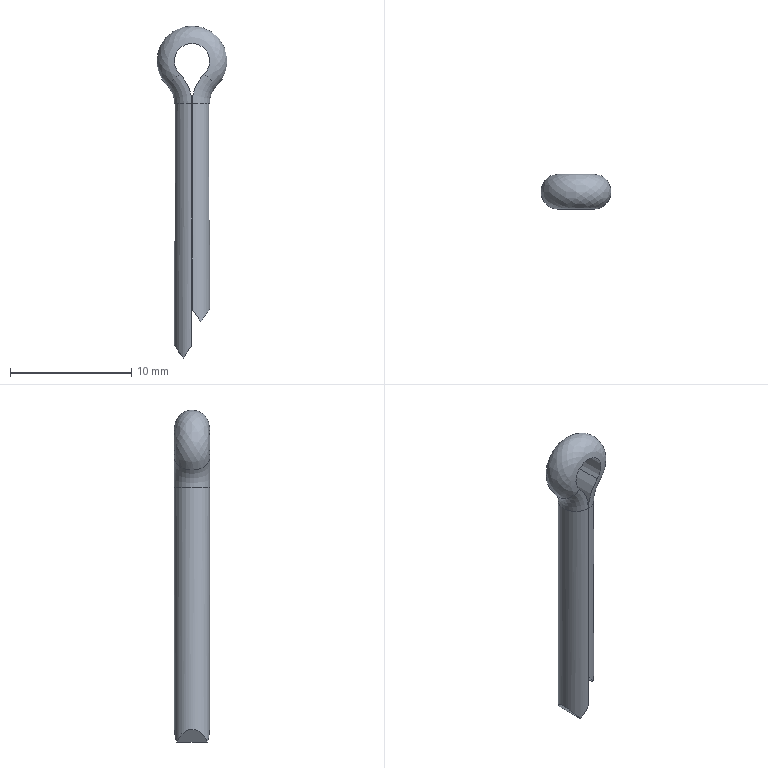Component | NX | 9 | 1 solid | 14 faces | box 5.8 x 2.9 x 27.4 mm | volume 172 mm3 | plane 6 | cylinder 5 | torus 2 | spline 1 | commonest cylinder face diameters 2.9 x2 6.988 x2 2.91 x1
STEP:
#1=CARTESIAN_POINT('',(0.,0.,0.));
#2=DIRECTION('',(0.,0.,1.));
#3=DIRECTION('',(1.,0.,0.));
#4=AXIS2_PLACEMENT_3D('',#1,#2,#3);
#5=CARTESIAN_POINT('',(-12.227,-1.254,0.6));
#6=VERTEX_POINT('',#5);
#7=CARTESIAN_POINT('',(-12.227,1.254,0.6));
#8=VERTEX_POINT('',#7);
#9=CARTESIAN_POINT('',(-12.227,-1.254,0.6));
#10=CARTESIAN_POINT('',(-12.95,-0.8352,1.632));
#11=CARTESIAN_POINT('',(-12.95,0.,1.632));
#12=CARTESIAN_POINT('',(-12.95,0.8352,1.632));
#13=CARTESIAN_POINT('',(-12.227,1.254,0.6));
#14=(BOUNDED_CURVE()B_SPLINE_CURVE(2,(#9,#10,#11,#12,#13),.UNSPECIFIED.,.F.,.F.)B_SPLINE_CURVE_WITH_KNOTS((3,2,3),(0.,0.5,1.),.PIECEWISE_BEZIER_KNOTS.)CURVE()GEOMETRIC_REPRESENTATION_ITEM()RATIONAL_B_SPLINE_CURVE((0.8689,0.8077,1.,0.8077,0.8689))REPRESENTATION_ITEM(''));
#15=CARTESIAN_POINT('',(-12.589,0.,1.116));
#16=DIRECTION('',(0.8192,0.,0.5736));
#17=DIRECTION('',(-0.5736,0.,0.8192));
#18=AXIS2_PLACEMENT_3D('',#15,#16,#17);
#19=PLANE('',#18);
#20=CARTESIAN_POINT('',(-0.6298,1.254));
#21=CARTESIAN_POINT('',(0.6298,0.8352));
#22=CARTESIAN_POINT('',(0.6298,-0.));
#23=CARTESIAN_POINT('',(0.6298,-0.8352));
#24=CARTESIAN_POINT('',(-0.6298,-1.254));
#25=(BOUNDED_CURVE()B_SPLINE_CURVE(2,(#20,#21,#22,#23,#24),.UNSPECIFIED.,.F.,.F.)B_SPLINE_CURVE_WITH_KNOTS((3,2,3),(0.,0.5,1.),.PIECEWISE_BEZIER_KNOTS.)CURVE()GEOMETRIC_REPRESENTATION_ITEM()RATIONAL_B_SPLINE_CURVE((0.8689,0.8077,1.,0.8077,0.8689))REPRESENTATION_ITEM(''));
#26=(GEOMETRIC_REPRESENTATION_CONTEXT(2)PARAMETRIC_REPRESENTATION_CONTEXT()REPRESENTATION_CONTEXT('',''));
#27=DEFINITIONAL_REPRESENTATION('',(#25),#26);
#28=PCURVE('',#19,#27);
#29=CARTESIAN_POINT('',(-11.5,0.,21.6));
#30=DIRECTION('',(0.,0.,-1.));
#31=DIRECTION('',(-0.003448,1.,-0.));
#32=AXIS2_PLACEMENT_3D('',#29,#30,#31);
#33=CYLINDRICAL_SURFACE('',#32,1.45);
#34=CARTESIAN_POINT('',(3.671,21.));
#35=CARTESIAN_POINT('',(3.703,20.942));
#36=CARTESIAN_POINT('',(3.768,20.828));
#37=CARTESIAN_POINT('',(3.867,20.668));
#38=CARTESIAN_POINT('',(3.966,20.521));
#39=CARTESIAN_POINT('',(4.065,20.389));
#40=CARTESIAN_POINT('',(4.163,20.273));
#41=CARTESIAN_POINT('',(4.261,20.176));
#42=CARTESIAN_POINT('',(4.356,20.098));
#43=CARTESIAN_POINT('',(4.45,20.038));
#44=CARTESIAN_POINT('',(4.541,19.997));
#45=CARTESIAN_POINT('',(4.63,19.973));
#46=CARTESIAN_POINT('',(4.716,19.966));
#47=CARTESIAN_POINT('',(4.801,19.973));
#48=CARTESIAN_POINT('',(4.89,19.997));
#49=CARTESIAN_POINT('',(4.982,20.038));
#50=CARTESIAN_POINT('',(5.075,20.098));
#51=CARTESIAN_POINT('',(5.171,20.176));
#52=CARTESIAN_POINT('',(5.268,20.273));
#53=CARTESIAN_POINT('',(5.366,20.389));
#54=CARTESIAN_POINT('',(5.465,20.521));
#55=CARTESIAN_POINT('',(5.564,20.668));
#56=CARTESIAN_POINT('',(5.663,20.828));
#57=CARTESIAN_POINT('',(5.729,20.942));
#58=CARTESIAN_POINT('',(5.761,21.));
#59=B_SPLINE_CURVE_WITH_KNOTS('',3,(#34,#35,#36,#37,#38,#39,#40,#41,#42,#43,#44,#45,#46,#47,#48,#49,#50,#51,#52,#53,#54,#55,#56,#57,#58),.UNSPECIFIED.,.F.,.F.,(4,1,1,1,1,1,1,1,1,1,1,1,1,1,1,1,1,1,1,1,1,1,4),(0.,0.04545,0.09091,0.1364,0.1818,0.2273,0.2727,0.3182,0.3636,0.4091,0.4545,0.5,0.5455,0.5909,0.6364,0.6818,0.7273,0.7727,0.8182,0.8636,0.9091,0.9545,1.),.QUASI_UNIFORM_KNOTS.);
#60=(GEOMETRIC_REPRESENTATION_CONTEXT(2)PARAMETRIC_REPRESENTATION_CONTEXT()REPRESENTATION_CONTEXT('',''));
#61=DEFINITIONAL_REPRESENTATION('',(#59),#60);
#62=PCURVE('',#33,#61);
#63=SURFACE_CURVE('',#14,(#28,#62),.PCURVE_S1.);
#64=EDGE_CURVE('',#6,#8,#63,.T.);
#65=ORIENTED_EDGE('',*,*,#64,.T.);
#66=CARTESIAN_POINT('',(-12.227,1.254,0.6));
#67=DIRECTION('',(0.,-1.,0.));
#68=VECTOR('',#67,1.);
#69=LINE('',#66,#68);
#70=CARTESIAN_POINT('',(-0.6298,-1.254));
#71=DIRECTION('',(0.,1.));
#72=VECTOR('',#71,1.);
#73=LINE('',#70,#72);
#74=(GEOMETRIC_REPRESENTATION_CONTEXT(2)PARAMETRIC_REPRESENTATION_CONTEXT()REPRESENTATION_CONTEXT('',''));
#75=DEFINITIONAL_REPRESENTATION('',(#73),#74);
#76=PCURVE('',#19,#75);
#77=CARTESIAN_POINT('',(-11.866,0.,1.116));
#78=DIRECTION('',(-0.8192,0.,0.5736));
#79=DIRECTION('',(-0.5736,0.,-0.8192));
#80=AXIS2_PLACEMENT_3D('',#77,#78,#79);
#81=PLANE('',#80);
#82=CARTESIAN_POINT('',(0.6298,-1.254));
#83=DIRECTION('',(0.,1.));
#84=VECTOR('',#83,1.);
#85=LINE('',#82,#84);
#86=(GEOMETRIC_REPRESENTATION_CONTEXT(2)PARAMETRIC_REPRESENTATION_CONTEXT()REPRESENTATION_CONTEXT('',''));
#87=DEFINITIONAL_REPRESENTATION('',(#85),#86);
#88=PCURVE('',#81,#87);
#89=SURFACE_CURVE('',#69,(#76,#88),.PCURVE_S1.);
#90=EDGE_CURVE('',#8,#6,#89,.T.);
#91=ORIENTED_EDGE('',*,*,#90,.T.);
#92=EDGE_LOOP('',(#65,#91));
#93=FACE_BOUND('',#92,.T.);
#94=ADVANCED_FACE('',(#93),#19,.F.);
#95=CARTESIAN_POINT('',(-11.505,1.45,1.632));
#96=VERTEX_POINT('',#95);
#97=CARTESIAN_POINT('',(-11.5,0.,1.639));
#98=DIRECTION('',(0.8192,0.,-0.5736));
#99=DIRECTION('',(-0.5736,-0.,-0.8192));
#100=AXIS2_PLACEMENT_3D('',#97,#98,#99);
#101=ELLIPSE('',#100,2.528,1.45);
#102=CARTESIAN_POINT('',(1.889,-0.));
#103=CARTESIAN_POINT('',(1.889,-2.511));
#104=CARTESIAN_POINT('',(-1.903,-1.256));
#105=CARTESIAN_POINT('',(-5.695,-0.));
#106=CARTESIAN_POINT('',(-1.903,1.256));
#107=CARTESIAN_POINT('',(1.889,2.511));
#108=CARTESIAN_POINT('',(1.889,-0.));
#109=(BOUNDED_CURVE()B_SPLINE_CURVE(2,(#102,#103,#104,#105,#106,#107,#108),.UNSPECIFIED.,.T.,.F.)B_SPLINE_CURVE_WITH_KNOTS((1,2,2,2,2,1),(-2.094,0.,2.094,4.189,6.283,8.378),.UNSPECIFIED.)CURVE()GEOMETRIC_REPRESENTATION_ITEM()RATIONAL_B_SPLINE_CURVE((1.,0.5,1.,0.5,1.,0.5,1.))REPRESENTATION_ITEM(''));
#110=(GEOMETRIC_REPRESENTATION_CONTEXT(2)PARAMETRIC_REPRESENTATION_CONTEXT()REPRESENTATION_CONTEXT('',''));
#111=DEFINITIONAL_REPRESENTATION('',(#109),#110);
#112=PCURVE('',#81,#111);
#113=CARTESIAN_POINT('',(5.761,21.));
#114=CARTESIAN_POINT('',(6.283,19.968));
#115=B_SPLINE_CURVE_WITH_KNOTS('',1,(#113,#114),.UNSPECIFIED.,.F.,.F.,(2,2),(1.045,1.567),.PIECEWISE_BEZIER_KNOTS.);
#116=(GEOMETRIC_REPRESENTATION_CONTEXT(2)PARAMETRIC_REPRESENTATION_CONTEXT()REPRESENTATION_CONTEXT('',''));
#117=DEFINITIONAL_REPRESENTATION('',(#115),#116);
#118=PCURVE('',#33,#117);
#119=SURFACE_CURVE('',#101,(#112,#118),.PCURVE_S1.);
#120=EDGE_CURVE('',#8,#96,#119,.T.);
#121=ORIENTED_EDGE('',*,*,#120,.T.);
#122=CARTESIAN_POINT('',(-11.505,-1.45,1.632));
#123=VERTEX_POINT('',#122);
#124=CARTESIAN_POINT('',(-11.505,1.45,1.632));
#125=DIRECTION('',(0.,-1.,0.));
#126=VECTOR('',#125,1.);
#127=LINE('',#124,#126);
#128=CARTESIAN_POINT('',(-0.6298,-1.45));
#129=DIRECTION('',(0.,1.));
#130=VECTOR('',#129,1.);
#131=LINE('',#128,#130);
#132=(GEOMETRIC_REPRESENTATION_CONTEXT(2)PARAMETRIC_REPRESENTATION_CONTEXT()REPRESENTATION_CONTEXT('',''));
#133=DEFINITIONAL_REPRESENTATION('',(#131),#132);
#134=PCURVE('',#81,#133);
#135=CARTESIAN_POINT('',(-11.505,0.,11.1));
#136=DIRECTION('',(-1.,-0.,-0.));
#137=DIRECTION('',(-0.,1.,-0.));
#138=AXIS2_PLACEMENT_3D('',#135,#136,#137);
#139=PLANE('',#138);
#140=CARTESIAN_POINT('',(1.45,9.468));
#141=DIRECTION('',(-1.,0.));
#142=VECTOR('',#141,1.);
#143=LINE('',#140,#142);
#144=(GEOMETRIC_REPRESENTATION_CONTEXT(2)PARAMETRIC_REPRESENTATION_CONTEXT()REPRESENTATION_CONTEXT('',''));
#145=DEFINITIONAL_REPRESENTATION('',(#143),#144);
#146=PCURVE('',#139,#145);
#147=SURFACE_CURVE('',#127,(#134,#146),.PCURVE_S1.);
#148=EDGE_CURVE('',#96,#123,#147,.T.);
#149=ORIENTED_EDGE('',*,*,#148,.T.);
#150=CARTESIAN_POINT('',(-11.5,0.,1.639));
#151=DIRECTION('',(0.8192,-0.,-0.5736));
#152=DIRECTION('',(-0.5736,-0.,-0.8192));
#153=AXIS2_PLACEMENT_3D('',#150,#151,#152);
#154=ELLIPSE('',#153,2.528,1.45);
#155=CARTESIAN_POINT('',(1.889,-0.));
#156=CARTESIAN_POINT('',(1.889,-2.511));
#157=CARTESIAN_POINT('',(-1.903,-1.256));
#158=CARTESIAN_POINT('',(-5.695,-0.));
#159=CARTESIAN_POINT('',(-1.903,1.256));
#160=CARTESIAN_POINT('',(1.889,2.511));
#161=CARTESIAN_POINT('',(1.889,-0.));
#162=(BOUNDED_CURVE()B_SPLINE_CURVE(2,(#155,#156,#157,#158,#159,#160,#161),.UNSPECIFIED.,.T.,.F.)B_SPLINE_CURVE_WITH_KNOTS((1,2,2,2,2,1),(-2.094,0.,2.094,4.189,6.283,8.378),.UNSPECIFIED.)CURVE()GEOMETRIC_REPRESENTATION_ITEM()RATIONAL_B_SPLINE_CURVE((1.,0.5,1.,0.5,1.,0.5,1.))REPRESENTATION_ITEM(''));
#163=(GEOMETRIC_REPRESENTATION_CONTEXT(2)PARAMETRIC_REPRESENTATION_CONTEXT()REPRESENTATION_CONTEXT('',''));
#164=DEFINITIONAL_REPRESENTATION('',(#162),#163);
#165=PCURVE('',#81,#164);
#166=CARTESIAN_POINT('',(3.148,19.968));
#167=CARTESIAN_POINT('',(3.671,21.));
#168=B_SPLINE_CURVE_WITH_KNOTS('',1,(#166,#167),.UNSPECIFIED.,.F.,.F.,(2,2),(4.716,5.238),.PIECEWISE_BEZIER_KNOTS.);
#169=(GEOMETRIC_REPRESENTATION_CONTEXT(2)PARAMETRIC_REPRESENTATION_CONTEXT()REPRESENTATION_CONTEXT('',''));
#170=DEFINITIONAL_REPRESENTATION('',(#168),#169);
#171=PCURVE('',#33,#170);
#172=SURFACE_CURVE('',#154,(#165,#171),.PCURVE_S1.);
#173=EDGE_CURVE('',#123,#6,#172,.T.);
#174=ORIENTED_EDGE('',*,*,#173,.T.);
#175=ORIENTED_EDGE('',*,*,#90,.F.);
#176=EDGE_LOOP('',(#121,#149,#174,#175));
#177=FACE_BOUND('',#176,.T.);
#178=ADVANCED_FACE('',(#177),#81,.F.);
#179=CARTESIAN_POINT('',(-10.773,1.254,3.6));
#180=VERTEX_POINT('',#179);
#181=CARTESIAN_POINT('',(-10.773,-1.254,3.6));
#182=VERTEX_POINT('',#181);
#183=CARTESIAN_POINT('',(-10.773,1.254,3.6));
#184=CARTESIAN_POINT('',(-10.05,0.8352,4.632));
#185=CARTESIAN_POINT('',(-10.05,0.,4.632));
#186=CARTESIAN_POINT('',(-10.05,-0.8352,4.632));
#187=CARTESIAN_POINT('',(-10.773,-1.254,3.6));
#188=(BOUNDED_CURVE()B_SPLINE_CURVE(2,(#183,#184,#185,#186,#187),.UNSPECIFIED.,.F.,.F.)B_SPLINE_CURVE_WITH_KNOTS((3,2,3),(0.,0.5,1.),.PIECEWISE_BEZIER_KNOTS.)CURVE()GEOMETRIC_REPRESENTATION_ITEM()RATIONAL_B_SPLINE_CURVE((0.8689,0.8077,1.,0.8077,0.8689))REPRESENTATION_ITEM(''));
#189=CARTESIAN_POINT('',(-10.411,0.,4.116));
#190=DIRECTION('',(-0.8192,0.,0.5736));
#191=DIRECTION('',(-0.5736,0.,-0.8192));
#192=AXIS2_PLACEMENT_3D('',#189,#190,#191);
#193=PLANE('',#192);
#194=CARTESIAN_POINT('',(0.6298,-1.254));
#195=CARTESIAN_POINT('',(-0.6298,-0.8352));
#196=CARTESIAN_POINT('',(-0.6298,-0.));
#197=CARTESIAN_POINT('',(-0.6298,0.8352));
#198=CARTESIAN_POINT('',(0.6298,1.254));
#199=(BOUNDED_CURVE()B_SPLINE_CURVE(2,(#194,#195,#196,#197,#198),.UNSPECIFIED.,.F.,.F.)B_SPLINE_CURVE_WITH_KNOTS((3,2,3),(0.,0.5,1.),.PIECEWISE_BEZIER_KNOTS.)CURVE()GEOMETRIC_REPRESENTATION_ITEM()RATIONAL_B_SPLINE_CURVE((0.8689,0.8077,1.,0.8077,0.8689))REPRESENTATION_ITEM(''));
#200=(GEOMETRIC_REPRESENTATION_CONTEXT(2)PARAMETRIC_REPRESENTATION_CONTEXT()REPRESENTATION_CONTEXT('',''));
#201=DEFINITIONAL_REPRESENTATION('',(#199),#200);
#202=PCURVE('',#193,#201);
#203=CARTESIAN_POINT('',(-11.5,0.,3.6));
#204=DIRECTION('',(-0.,0.,1.));
#205=DIRECTION('',(0.003448,1.,0.));
#206=AXIS2_PLACEMENT_3D('',#203,#204,#205);
#207=CYLINDRICAL_SURFACE('',#206,1.45);
#208=CARTESIAN_POINT('',(5.761,-0.));
#209=CARTESIAN_POINT('',(5.729,0.05815));
#210=CARTESIAN_POINT('',(5.663,0.1718));
#211=CARTESIAN_POINT('',(5.564,0.3321));
#212=CARTESIAN_POINT('',(5.465,0.4793));
#213=CARTESIAN_POINT('',(5.366,0.6114));
#214=CARTESIAN_POINT('',(5.268,0.7267));
#215=CARTESIAN_POINT('',(5.171,0.8239));
#216=CARTESIAN_POINT('',(5.075,0.9023));
#217=CARTESIAN_POINT('',(4.982,0.9619));
#218=CARTESIAN_POINT('',(4.89,1.003));
#219=CARTESIAN_POINT('',(4.801,1.027));
#220=CARTESIAN_POINT('',(4.716,1.034));
#221=CARTESIAN_POINT('',(4.63,1.027));
#222=CARTESIAN_POINT('',(4.541,1.003));
#223=CARTESIAN_POINT('',(4.45,0.9619));
#224=CARTESIAN_POINT('',(4.356,0.9023));
#225=CARTESIAN_POINT('',(4.261,0.8239));
#226=CARTESIAN_POINT('',(4.163,0.7267));
#227=CARTESIAN_POINT('',(4.065,0.6114));
#228=CARTESIAN_POINT('',(3.966,0.4793));
#229=CARTESIAN_POINT('',(3.867,0.3321));
#230=CARTESIAN_POINT('',(3.768,0.1718));
#231=CARTESIAN_POINT('',(3.703,0.05815));
#232=CARTESIAN_POINT('',(3.671,-0.));
#233=B_SPLINE_CURVE_WITH_KNOTS('',3,(#208,#209,#210,#211,#212,#213,#214,#215,#216,#217,#218,#219,#220,#221,#222,#223,#224,#225,#226,#227,#228,#229,#230,#231,#232),.UNSPECIFIED.,.F.,.F.,(4,1,1,1,1,1,1,1,1,1,1,1,1,1,1,1,1,1,1,1,1,1,4),(0.,0.04545,0.09091,0.1364,0.1818,0.2273,0.2727,0.3182,0.3636,0.4091,0.4545,0.5,0.5455,0.5909,0.6364,0.6818,0.7273,0.7727,0.8182,0.8636,0.9091,0.9545,1.),.QUASI_UNIFORM_KNOTS.);
#234=(GEOMETRIC_REPRESENTATION_CONTEXT(2)PARAMETRIC_REPRESENTATION_CONTEXT()REPRESENTATION_CONTEXT('',''));
#235=DEFINITIONAL_REPRESENTATION('',(#233),#234);
#236=PCURVE('',#207,#235);
#237=SURFACE_CURVE('',#188,(#202,#236),.PCURVE_S1.);
#238=EDGE_CURVE('',#180,#182,#237,.T.);
#239=ORIENTED_EDGE('',*,*,#238,.T.);
#240=CARTESIAN_POINT('',(-10.773,1.254,3.6));
#241=DIRECTION('',(0.,-1.,0.));
#242=VECTOR('',#241,1.);
#243=LINE('',#240,#242);
#244=CARTESIAN_POINT('',(0.6298,-1.254));
#245=DIRECTION('',(0.,1.));
#246=VECTOR('',#245,1.);
#247=LINE('',#244,#246);
#248=(GEOMETRIC_REPRESENTATION_CONTEXT(2)PARAMETRIC_REPRESENTATION_CONTEXT()REPRESENTATION_CONTEXT('',''));
#249=DEFINITIONAL_REPRESENTATION('',(#247),#248);
#250=PCURVE('',#193,#249);
#251=CARTESIAN_POINT('',(-11.134,0.,4.116));
#252=DIRECTION('',(0.8192,0.,0.5736));
#253=DIRECTION('',(-0.5736,0.,0.8192));
#254=AXIS2_PLACEMENT_3D('',#251,#252,#253);
#255=PLANE('',#254);
#256=CARTESIAN_POINT('',(-0.6298,-1.254));
#257=DIRECTION('',(0.,1.));
#258=VECTOR('',#257,1.);
#259=LINE('',#256,#258);
#260=(GEOMETRIC_REPRESENTATION_CONTEXT(2)PARAMETRIC_REPRESENTATION_CONTEXT()REPRESENTATION_CONTEXT('',''));
#261=DEFINITIONAL_REPRESENTATION('',(#259),#260);
#262=PCURVE('',#255,#261);
#263=SURFACE_CURVE('',#243,(#250,#262),.PCURVE_S1.);
#264=EDGE_CURVE('',#180,#182,#263,.T.);
#265=ORIENTED_EDGE('',*,*,#264,.F.);
#266=EDGE_LOOP('',(#239,#265));
#267=FACE_BOUND('',#266,.T.);
#268=ADVANCED_FACE('',(#267),#193,.F.);
#269=CARTESIAN_POINT('',(-11.495,-1.45,4.632));
#270=VERTEX_POINT('',#269);
#271=CARTESIAN_POINT('',(-11.5,-0.,4.639));
#272=DIRECTION('',(-0.8192,-0.,-0.5736));
#273=DIRECTION('',(0.5736,0.,-0.8192));
#274=AXIS2_PLACEMENT_3D('',#271,#272,#273);
#275=ELLIPSE('',#274,2.528,1.45);
#276=CARTESIAN_POINT('',(-1.889,0.));
#277=CARTESIAN_POINT('',(-1.889,2.511));
#278=CARTESIAN_POINT('',(1.903,1.256));
#279=CARTESIAN_POINT('',(5.695,0.));
#280=CARTESIAN_POINT('',(1.903,-1.256));
#281=CARTESIAN_POINT('',(-1.889,-2.511));
#282=CARTESIAN_POINT('',(-1.889,0.));
#283=(BOUNDED_CURVE()B_SPLINE_CURVE(2,(#276,#277,#278,#279,#280,#281,#282),.UNSPECIFIED.,.T.,.F.)B_SPLINE_CURVE_WITH_KNOTS((1,2,2,2,2,1),(-2.094,0.,2.094,4.189,6.283,8.378),.UNSPECIFIED.)CURVE()GEOMETRIC_REPRESENTATION_ITEM()RATIONAL_B_SPLINE_CURVE((1.,0.5,1.,0.5,1.,0.5,1.))REPRESENTATION_ITEM(''));
#284=(GEOMETRIC_REPRESENTATION_CONTEXT(2)PARAMETRIC_REPRESENTATION_CONTEXT()REPRESENTATION_CONTEXT('',''));
#285=DEFINITIONAL_REPRESENTATION('',(#283),#284);
#286=PCURVE('',#255,#285);
#287=CARTESIAN_POINT('',(3.671,0.));
#288=CARTESIAN_POINT('',(3.148,1.032));
#289=B_SPLINE_CURVE_WITH_KNOTS('',1,(#287,#288),.UNSPECIFIED.,.F.,.F.,(2,2),(1.045,1.567),.PIECEWISE_BEZIER_KNOTS.);
#290=(GEOMETRIC_REPRESENTATION_CONTEXT(2)PARAMETRIC_REPRESENTATION_CONTEXT()REPRESENTATION_CONTEXT('',''));
#291=DEFINITIONAL_REPRESENTATION('',(#289),#290);
#292=PCURVE('',#207,#291);
#293=SURFACE_CURVE('',#275,(#286,#292),.PCURVE_S1.);
#294=EDGE_CURVE('',#182,#270,#293,.T.);
#295=ORIENTED_EDGE('',*,*,#294,.T.);
#296=CARTESIAN_POINT('',(-11.495,1.45,4.632));
#297=VERTEX_POINT('',#296);
#298=CARTESIAN_POINT('',(-11.495,1.45,4.632));
#299=DIRECTION('',(0.,-1.,0.));
#300=VECTOR('',#299,1.);
#301=LINE('',#298,#300);
#302=CARTESIAN_POINT('',(0.6298,-1.45));
#303=DIRECTION('',(0.,1.));
#304=VECTOR('',#303,1.);
#305=LINE('',#302,#304);
#306=(GEOMETRIC_REPRESENTATION_CONTEXT(2)PARAMETRIC_REPRESENTATION_CONTEXT()REPRESENTATION_CONTEXT('',''));
#307=DEFINITIONAL_REPRESENTATION('',(#305),#306);
#308=PCURVE('',#255,#307);
#309=CARTESIAN_POINT('',(-11.495,0.,12.6));
#310=DIRECTION('',(1.,-0.,0.));
#311=DIRECTION('',(0.,1.,0.));
#312=AXIS2_PLACEMENT_3D('',#309,#310,#311);
#313=PLANE('',#312);
#314=CARTESIAN_POINT('',(1.45,-7.968));
#315=DIRECTION('',(-1.,-0.));
#316=VECTOR('',#315,1.);
#317=LINE('',#314,#316);
#318=(GEOMETRIC_REPRESENTATION_CONTEXT(2)PARAMETRIC_REPRESENTATION_CONTEXT()REPRESENTATION_CONTEXT('',''));
#319=DEFINITIONAL_REPRESENTATION('',(#317),#318);
#320=PCURVE('',#313,#319);
#321=SURFACE_CURVE('',#301,(#308,#320),.PCURVE_S1.);
#322=EDGE_CURVE('',#297,#270,#321,.T.);
#323=ORIENTED_EDGE('',*,*,#322,.F.);
#324=CARTESIAN_POINT('',(-11.5,-0.,4.639));
#325=DIRECTION('',(-0.8192,0.,-0.5736));
#326=DIRECTION('',(0.5736,0.,-0.8192));
#327=AXIS2_PLACEMENT_3D('',#324,#325,#326);
#328=ELLIPSE('',#327,2.528,1.45);
#329=CARTESIAN_POINT('',(-1.889,0.));
#330=CARTESIAN_POINT('',(-1.889,2.511));
#331=CARTESIAN_POINT('',(1.903,1.256));
#332=CARTESIAN_POINT('',(5.695,0.));
#333=CARTESIAN_POINT('',(1.903,-1.256));
#334=CARTESIAN_POINT('',(-1.889,-2.511));
#335=CARTESIAN_POINT('',(-1.889,0.));
#336=(BOUNDED_CURVE()B_SPLINE_CURVE(2,(#329,#330,#331,#332,#333,#334,#335),.UNSPECIFIED.,.T.,.F.)B_SPLINE_CURVE_WITH_KNOTS((1,2,2,2,2,1),(-2.094,0.,2.094,4.189,6.283,8.378),.UNSPECIFIED.)CURVE()GEOMETRIC_REPRESENTATION_ITEM()RATIONAL_B_SPLINE_CURVE((1.,0.5,1.,0.5,1.,0.5,1.))REPRESENTATION_ITEM(''));
#337=(GEOMETRIC_REPRESENTATION_CONTEXT(2)PARAMETRIC_REPRESENTATION_CONTEXT()REPRESENTATION_CONTEXT('',''));
#338=DEFINITIONAL_REPRESENTATION('',(#336),#337);
#339=PCURVE('',#255,#338);
#340=CARTESIAN_POINT('',(6.283,1.032));
#341=CARTESIAN_POINT('',(5.761,0.));
#342=B_SPLINE_CURVE_WITH_KNOTS('',1,(#340,#341),.UNSPECIFIED.,.F.,.F.,(2,2),(4.716,5.238),.PIECEWISE_BEZIER_KNOTS.);
#343=(GEOMETRIC_REPRESENTATION_CONTEXT(2)PARAMETRIC_REPRESENTATION_CONTEXT()REPRESENTATION_CONTEXT('',''));
#344=DEFINITIONAL_REPRESENTATION('',(#342),#343);
#345=PCURVE('',#207,#344);
#346=SURFACE_CURVE('',#328,(#339,#345),.PCURVE_S1.);
#347=EDGE_CURVE('',#297,#180,#346,.T.);
#348=ORIENTED_EDGE('',*,*,#347,.T.);
#349=ORIENTED_EDGE('',*,*,#264,.T.);
#350=EDGE_LOOP('',(#295,#323,#348,#349));
#351=FACE_BOUND('',#350,.T.);
#352=ADVANCED_FACE('',(#351),#255,.F.);
#353=CARTESIAN_POINT('',(-11.505,-1.45,21.6));
#354=VERTEX_POINT('',#353);
#355=CARTESIAN_POINT('',(-11.505,-1.45,21.6));
#356=DIRECTION('',(0.,0.,-1.));
#357=VECTOR('',#356,1.);
#358=LINE('',#355,#357);
#359=CARTESIAN_POINT('',(-1.45,-10.5));
#360=DIRECTION('',(0.,1.));
#361=VECTOR('',#360,1.);
#362=LINE('',#359,#361);
#363=(GEOMETRIC_REPRESENTATION_CONTEXT(2)PARAMETRIC_REPRESENTATION_CONTEXT()REPRESENTATION_CONTEXT('',''));
#364=DEFINITIONAL_REPRESENTATION('',(#362),#363);
#365=PCURVE('',#139,#364);
#366=CARTESIAN_POINT('',(3.148,0.));
#367=DIRECTION('',(0.,1.));
#368=VECTOR('',#367,1.);
#369=LINE('',#366,#368);
#370=(GEOMETRIC_REPRESENTATION_CONTEXT(2)PARAMETRIC_REPRESENTATION_CONTEXT()REPRESENTATION_CONTEXT('',''));
#371=DEFINITIONAL_REPRESENTATION('',(#369),#370);
#372=PCURVE('',#33,#371);
#373=SURFACE_CURVE('',#358,(#365,#372),.PCURVE_S1.);
#374=EDGE_CURVE('',#354,#123,#373,.T.);
#375=ORIENTED_EDGE('',*,*,#374,.T.);
#376=ORIENTED_EDGE('',*,*,#148,.F.);
#377=CARTESIAN_POINT('',(-11.505,1.45,21.6));
#378=VERTEX_POINT('',#377);
#379=CARTESIAN_POINT('',(-11.505,1.45,21.6));
#380=DIRECTION('',(-0.,0.,1.));
#381=VECTOR('',#380,1.);
#382=LINE('',#379,#381);
#383=CARTESIAN_POINT('',(1.45,-10.5));
#384=DIRECTION('',(-0.,-1.));
#385=VECTOR('',#384,1.);
#386=LINE('',#383,#385);
#387=(GEOMETRIC_REPRESENTATION_CONTEXT(2)PARAMETRIC_REPRESENTATION_CONTEXT()REPRESENTATION_CONTEXT('',''));
#388=DEFINITIONAL_REPRESENTATION('',(#386),#387);
#389=PCURVE('',#139,#388);
#390=CARTESIAN_POINT('',(6.283,0.));
#391=DIRECTION('',(0.,-1.));
#392=VECTOR('',#391,1.);
#393=LINE('',#390,#392);
#394=(GEOMETRIC_REPRESENTATION_CONTEXT(2)PARAMETRIC_REPRESENTATION_CONTEXT()REPRESENTATION_CONTEXT('',''));
#395=DEFINITIONAL_REPRESENTATION('',(#393),#394);
#396=PCURVE('',#33,#395);
#397=SURFACE_CURVE('',#382,(#389,#396),.PCURVE_S1.);
#398=EDGE_CURVE('',#96,#378,#397,.T.);
#399=ORIENTED_EDGE('',*,*,#398,.T.);
#400=CARTESIAN_POINT('',(-11.505,-1.45,21.6));
#401=DIRECTION('',(-0.,1.,-0.));
#402=VECTOR('',#401,1.);
#403=LINE('',#400,#402);
#404=CARTESIAN_POINT('',(-1.45,-10.5));
#405=DIRECTION('',(1.,0.));
#406=VECTOR('',#405,1.);
#407=LINE('',#404,#406);
#408=(GEOMETRIC_REPRESENTATION_CONTEXT(2)PARAMETRIC_REPRESENTATION_CONTEXT()REPRESENTATION_CONTEXT('',''));
#409=DEFINITIONAL_REPRESENTATION('',(#407),#408);
#410=PCURVE('',#139,#409);
#411=CARTESIAN_POINT('',(-14.999,-1.45,21.6));
#412=DIRECTION('',(0.,1.,-0.));
#413=DIRECTION('',(0.707,0.,0.7072));
#414=AXIS2_PLACEMENT_3D('',#411,#412,#413);
#415=CYLINDRICAL_SURFACE('',#414,3.494);
#416=CARTESIAN_POINT('',(0.7855,0.));
#417=DIRECTION('',(0.,1.));
#418=VECTOR('',#417,1.);
#419=LINE('',#416,#418);
#420=(GEOMETRIC_REPRESENTATION_CONTEXT(2)PARAMETRIC_REPRESENTATION_CONTEXT()REPRESENTATION_CONTEXT('',''));
#421=DEFINITIONAL_REPRESENTATION('',(#419),#420);
#422=PCURVE('',#415,#421);
#423=SURFACE_CURVE('',#403,(#410,#422),.PCURVE_S1.);
#424=EDGE_CURVE('',#354,#378,#423,.T.);
#425=ORIENTED_EDGE('',*,*,#424,.F.);
#426=EDGE_LOOP('',(#375,#376,#399,#425));
#427=FACE_BOUND('',#426,.T.);
#428=ADVANCED_FACE('',(#427),#139,.F.);
#429=ORIENTED_EDGE('',*,*,#398,.F.);
#430=ORIENTED_EDGE('',*,*,#120,.F.);
#431=ORIENTED_EDGE('',*,*,#64,.F.);
#432=ORIENTED_EDGE('',*,*,#173,.F.);
#433=ORIENTED_EDGE('',*,*,#374,.F.);
#434=CARTESIAN_POINT('',(-11.5,0.,21.6));
#435=DIRECTION('',(0.,-0.,1.));
#436=DIRECTION('',(-0.003448,1.,0.));
#437=AXIS2_PLACEMENT_3D('',#434,#435,#436);
#438=CIRCLE('',#437,1.45);
#439=CARTESIAN_POINT('',(6.283,0.));
#440=DIRECTION('',(-1.,0.));
#441=VECTOR('',#440,1.);
#442=LINE('',#439,#441);
#443=(GEOMETRIC_REPRESENTATION_CONTEXT(2)PARAMETRIC_REPRESENTATION_CONTEXT()REPRESENTATION_CONTEXT('',''));
#444=DEFINITIONAL_REPRESENTATION('',(#442),#443);
#445=PCURVE('',#33,#444);
#446=CARTESIAN_POINT('',(-14.999,0.,21.6));
#447=DIRECTION('',(0.,-1.,0.));
#448=DIRECTION('',(0.707,0.,0.7072));
#449=AXIS2_PLACEMENT_3D('',#446,#447,#448);
#450=TOROIDAL_SURFACE('',#449,3.499,1.45);
#451=CARTESIAN_POINT('',(5.498,4.709));
#452=DIRECTION('',(0.,-1.));
#453=VECTOR('',#452,1.);
#454=LINE('',#451,#453);
#455=(GEOMETRIC_REPRESENTATION_CONTEXT(2)PARAMETRIC_REPRESENTATION_CONTEXT()REPRESENTATION_CONTEXT('',''));
#456=DEFINITIONAL_REPRESENTATION('',(#454),#455);
#457=PCURVE('',#450,#456);
#458=SURFACE_CURVE('',#438,(#445,#457),.PCURVE_S1.);
#459=EDGE_CURVE('',#378,#354,#458,.T.);
#460=ORIENTED_EDGE('',*,*,#459,.F.);
#461=EDGE_LOOP('',(#429,#430,#431,#432,#433,#460));
#462=FACE_BOUND('',#461,.T.);
#463=ADVANCED_FACE('',(#462),#33,.T.);
#464=ORIENTED_EDGE('',*,*,#424,.T.);
#465=CARTESIAN_POINT('',(-12.529,1.45,24.071));
#466=VERTEX_POINT('',#465);
#467=CARTESIAN_POINT('',(-14.999,1.45,21.6));
#468=DIRECTION('',(0.,-1.,0.));
#469=DIRECTION('',(0.707,0.,0.7072));
#470=AXIS2_PLACEMENT_3D('',#467,#468,#469);
#471=CIRCLE('',#470,3.494);
#472=CARTESIAN_POINT('',(6.283,2.9));
#473=DIRECTION('',(-1.,-0.));
#474=VECTOR('',#473,1.);
#475=LINE('',#472,#474);
#476=(GEOMETRIC_REPRESENTATION_CONTEXT(2)PARAMETRIC_REPRESENTATION_CONTEXT()REPRESENTATION_CONTEXT('',''));
#477=DEFINITIONAL_REPRESENTATION('',(#475),#476);
#478=PCURVE('',#415,#477);
#479=CARTESIAN_POINT('',(0.,4.709));
#480=DIRECTION('',(1.,0.));
#481=VECTOR('',#480,1.);
#482=LINE('',#479,#481);
#483=(GEOMETRIC_REPRESENTATION_CONTEXT(2)PARAMETRIC_REPRESENTATION_CONTEXT()REPRESENTATION_CONTEXT('',''));
#484=DEFINITIONAL_REPRESENTATION('',(#482),#483);
#485=PCURVE('',#450,#484);
#486=SURFACE_CURVE('',#471,(#478,#485),.PCURVE_S1.);
#487=EDGE_CURVE('',#378,#466,#486,.T.);
#488=ORIENTED_EDGE('',*,*,#487,.T.);
#489=CARTESIAN_POINT('',(-12.529,-1.45,24.071));
#490=VERTEX_POINT('',#489);
#491=CARTESIAN_POINT('',(-12.529,-1.45,24.071));
#492=DIRECTION('',(-0.,1.,0.));
#493=VECTOR('',#492,1.);
#494=LINE('',#491,#493);
#495=CARTESIAN_POINT('',(0.,-0.));
#496=DIRECTION('',(0.,1.));
#497=VECTOR('',#496,1.);
#498=LINE('',#495,#497);
#499=(GEOMETRIC_REPRESENTATION_CONTEXT(2)PARAMETRIC_REPRESENTATION_CONTEXT()REPRESENTATION_CONTEXT('',''));
#500=DEFINITIONAL_REPRESENTATION('',(#498),#499);
#501=PCURVE('',#415,#500);
#502=CARTESIAN_POINT('',(-11.5,-1.45,25.1));
#503=DIRECTION('',(0.,1.,-0.));
#504=DIRECTION('',(0.707,-0.,-0.7072));
#505=AXIS2_PLACEMENT_3D('',#502,#503,#504);
#506=CYLINDRICAL_SURFACE('',#505,1.455);
#507=CARTESIAN_POINT('',(1.571,0.));
#508=DIRECTION('',(0.,1.));
#509=VECTOR('',#508,1.);
#510=LINE('',#507,#509);
#511=(GEOMETRIC_REPRESENTATION_CONTEXT(2)PARAMETRIC_REPRESENTATION_CONTEXT()REPRESENTATION_CONTEXT('',''));
#512=DEFINITIONAL_REPRESENTATION('',(#510),#511);
#513=PCURVE('',#506,#512);
#514=SURFACE_CURVE('',#494,(#501,#513),.PCURVE_S1.);
#515=EDGE_CURVE('',#490,#466,#514,.T.);
#516=ORIENTED_EDGE('',*,*,#515,.F.);
#517=CARTESIAN_POINT('',(-14.999,-1.45,21.6));
#518=DIRECTION('',(0.,1.,0.));
#519=DIRECTION('',(0.707,-0.,0.7072));
#520=AXIS2_PLACEMENT_3D('',#517,#518,#519);
#521=CIRCLE('',#520,3.494);
#522=CARTESIAN_POINT('',(0.,-0.));
#523=DIRECTION('',(1.,0.));
#524=VECTOR('',#523,1.);
#525=LINE('',#522,#524);
#526=(GEOMETRIC_REPRESENTATION_CONTEXT(2)PARAMETRIC_REPRESENTATION_CONTEXT()REPRESENTATION_CONTEXT('',''));
#527=DEFINITIONAL_REPRESENTATION('',(#525),#526);
#528=PCURVE('',#415,#527);
#529=CARTESIAN_POINT('',(6.283,1.574));
#530=DIRECTION('',(-1.,0.));
#531=VECTOR('',#530,1.);
#532=LINE('',#529,#531);
#533=(GEOMETRIC_REPRESENTATION_CONTEXT(2)PARAMETRIC_REPRESENTATION_CONTEXT()REPRESENTATION_CONTEXT('',''));
#534=DEFINITIONAL_REPRESENTATION('',(#532),#533);
#535=PCURVE('',#450,#534);
#536=SURFACE_CURVE('',#521,(#528,#535),.PCURVE_S1.);
#537=EDGE_CURVE('',#490,#354,#536,.T.);
#538=ORIENTED_EDGE('',*,*,#537,.T.);
#539=EDGE_LOOP('',(#464,#488,#516,#538));
#540=FACE_BOUND('',#539,.T.);
#541=ADVANCED_FACE('',(#540),#415,.T.);
#542=ORIENTED_EDGE('',*,*,#459,.T.);
#543=ORIENTED_EDGE('',*,*,#537,.F.);
#544=CARTESIAN_POINT('',(-12.525,0.,24.075));
#545=DIRECTION('',(-0.7072,0.,0.707));
#546=DIRECTION('',(-0.002438,1.,-0.002439));
#547=AXIS2_PLACEMENT_3D('',#544,#545,#546);
#548=CIRCLE('',#547,1.45);
#549=CARTESIAN_POINT('',(6.283,4.709));
#550=DIRECTION('',(0.,-1.));
#551=VECTOR('',#550,1.);
#552=LINE('',#549,#551);
#553=(GEOMETRIC_REPRESENTATION_CONTEXT(2)PARAMETRIC_REPRESENTATION_CONTEXT()REPRESENTATION_CONTEXT('',''));
#554=DEFINITIONAL_REPRESENTATION('',(#552),#553);
#555=PCURVE('',#450,#554);
#556=CARTESIAN_POINT('',(-10.471,1.45,24.071));
#557=CARTESIAN_POINT('',(-9.784,1.45,24.758));
#558=CARTESIAN_POINT('',(-10.156,1.45,25.657));
#559=CARTESIAN_POINT('',(-10.528,1.45,26.555));
#560=CARTESIAN_POINT('',(-11.5,1.45,26.555));
#561=CARTESIAN_POINT('',(-12.472,1.45,26.555));
#562=CARTESIAN_POINT('',(-12.844,1.45,25.657));
#563=CARTESIAN_POINT('',(-13.216,1.45,24.758));
#564=CARTESIAN_POINT('',(-12.529,1.45,24.071));
#565=CARTESIAN_POINT('',(-9.45,1.445,23.049));
#566=CARTESIAN_POINT('',(-8.079,1.445,24.419));
#567=CARTESIAN_POINT('',(-8.821,1.445,26.21));
#568=CARTESIAN_POINT('',(-9.562,1.445,28.));
#569=CARTESIAN_POINT('',(-11.5,1.445,28.));
#570=CARTESIAN_POINT('',(-13.438,1.445,28.));
#571=CARTESIAN_POINT('',(-14.179,1.445,26.21));
#572=CARTESIAN_POINT('',(-14.921,1.445,24.419));
#573=CARTESIAN_POINT('',(-13.55,1.445,23.049));
#574=CARTESIAN_POINT('',(-9.45,0.,23.049));
#575=CARTESIAN_POINT('',(-8.079,0.,24.419));
#576=CARTESIAN_POINT('',(-8.821,0.,26.21));
#577=CARTESIAN_POINT('',(-9.562,0.,28.));
#578=CARTESIAN_POINT('',(-11.5,0.,28.));
#579=CARTESIAN_POINT('',(-13.438,0.,28.));
#580=CARTESIAN_POINT('',(-14.179,0.,26.21));
#581=CARTESIAN_POINT('',(-14.921,0.,24.419));
#582=CARTESIAN_POINT('',(-13.55,0.,23.049));
#583=CARTESIAN_POINT('',(-9.45,-1.445,23.049));
#584=CARTESIAN_POINT('',(-8.079,-1.445,24.419));
#585=CARTESIAN_POINT('',(-8.821,-1.445,26.21));
#586=CARTESIAN_POINT('',(-9.562,-1.445,28.));
#587=CARTESIAN_POINT('',(-11.5,-1.445,28.));
#588=CARTESIAN_POINT('',(-13.438,-1.445,28.));
#589=CARTESIAN_POINT('',(-14.179,-1.445,26.21));
#590=CARTESIAN_POINT('',(-14.921,-1.445,24.419));
#591=CARTESIAN_POINT('',(-13.55,-1.445,23.049));
#592=CARTESIAN_POINT('',(-10.471,-1.45,24.071));
#593=CARTESIAN_POINT('',(-9.784,-1.45,24.758));
#594=CARTESIAN_POINT('',(-10.156,-1.45,25.657));
#595=CARTESIAN_POINT('',(-10.528,-1.45,26.555));
#596=CARTESIAN_POINT('',(-11.5,-1.45,26.555));
#597=CARTESIAN_POINT('',(-12.472,-1.45,26.555));
#598=CARTESIAN_POINT('',(-12.844,-1.45,25.657));
#599=CARTESIAN_POINT('',(-13.216,-1.45,24.758));
#600=CARTESIAN_POINT('',(-12.529,-1.45,24.071));
#601=(BOUNDED_SURFACE()B_SPLINE_SURFACE(2,2,((#556,#557,#558,#559,#560,#561,#562,#563,#564),(#565,#566,#567,#568,#569,#570,#571,#572,#573),(#574,#575,#576,#577,#578,#579,#580,#581,#582),(#583,#584,#585,#586,#587,#588,#589,#590,#591),(#592,#593,#594,#595,#596,#597,#598,#599,#600)),.UNSPECIFIED.,.F.,.F.,.F.)B_SPLINE_SURFACE_WITH_KNOTS((3,2,3),(3,2,2,2,3),(0.,0.5,1.),(0.,0.25,0.5,0.75,1.),.PIECEWISE_BEZIER_KNOTS.)GEOMETRIC_REPRESENTATION_ITEM()RATIONAL_B_SPLINE_SURFACE(((1.,0.8315,1.,0.8315,1.,0.8315,1.,0.8315,1.),(0.7083,0.5889,0.7083,0.5889,0.7083,0.5889,0.7083,0.5889,0.7083),(1.,0.8315,1.,0.8315,1.,0.8315,1.,0.8315,1.),(0.7083,0.5889,0.7083,0.5889,0.7083,0.5889,0.7083,0.5889,0.7083),(1.,0.8315,1.,0.8315,1.,0.8315,1.,0.8315,1.)))REPRESENTATION_ITEM('')SURFACE());
#602=CARTESIAN_POINT('',(0.,1.));
#603=CARTESIAN_POINT('',(1.,1.));
#604=B_SPLINE_CURVE_WITH_KNOTS('',1,(#602,#603),.UNSPECIFIED.,.F.,.F.,(2,2),(0.,3.135),.PIECEWISE_BEZIER_KNOTS.);
#605=(GEOMETRIC_REPRESENTATION_CONTEXT(2)PARAMETRIC_REPRESENTATION_CONTEXT()REPRESENTATION_CONTEXT('',''));
#606=DEFINITIONAL_REPRESENTATION('',(#604),#605);
#607=PCURVE('',#601,#606);
#608=SURFACE_CURVE('',#548,(#555,#607),.PCURVE_S1.);
#609=EDGE_CURVE('',#466,#490,#608,.T.);
#610=ORIENTED_EDGE('',*,*,#609,.F.);
#611=ORIENTED_EDGE('',*,*,#487,.F.);
#612=EDGE_LOOP('',(#542,#543,#610,#611));
#613=FACE_BOUND('',#612,.T.);
#614=ADVANCED_FACE('',(#613),#450,.T.);
#615=CARTESIAN_POINT('',(-10.471,-1.45,24.071));
#616=VERTEX_POINT('',#615);
#617=CARTESIAN_POINT('',(-11.5,-1.45,25.1));
#618=DIRECTION('',(-0.,1.,0.));
#619=DIRECTION('',(0.707,0.,-0.7072));
#620=AXIS2_PLACEMENT_3D('',#617,#618,#619);
#621=CIRCLE('',#620,1.455);
#622=CARTESIAN_POINT('',(0.,-0.));
#623=DIRECTION('',(1.,0.));
#624=VECTOR('',#623,1.);
#625=LINE('',#622,#624);
#626=(GEOMETRIC_REPRESENTATION_CONTEXT(2)PARAMETRIC_REPRESENTATION_CONTEXT()REPRESENTATION_CONTEXT('',''));
#627=DEFINITIONAL_REPRESENTATION('',(#625),#626);
#628=PCURVE('',#506,#627);
#629=CARTESIAN_POINT('',(1.,1.));
#630=CARTESIAN_POINT('',(1.,-0.));
#631=B_SPLINE_CURVE_WITH_KNOTS('',1,(#629,#630),.UNSPECIFIED.,.F.,.F.,(2,2),(1.571,6.283),.PIECEWISE_BEZIER_KNOTS.);
#632=(GEOMETRIC_REPRESENTATION_CONTEXT(2)PARAMETRIC_REPRESENTATION_CONTEXT()REPRESENTATION_CONTEXT('',''));
#633=DEFINITIONAL_REPRESENTATION('',(#631),#632);
#634=PCURVE('',#601,#633);
#635=SURFACE_CURVE('',#621,(#628,#634),.PCURVE_S1.);
#636=EDGE_CURVE('',#490,#616,#635,.T.);
#637=ORIENTED_EDGE('',*,*,#636,.T.);
#638=CARTESIAN_POINT('',(-10.471,1.45,24.071));
#639=VERTEX_POINT('',#638);
#640=CARTESIAN_POINT('',(-10.471,-1.45,24.071));
#641=DIRECTION('',(0.,1.,-0.));
#642=VECTOR('',#641,1.);
#643=LINE('',#640,#642);
#644=CARTESIAN_POINT('',(6.283,0.));
#645=DIRECTION('',(0.,1.));
#646=VECTOR('',#645,1.);
#647=LINE('',#644,#646);
#648=(GEOMETRIC_REPRESENTATION_CONTEXT(2)PARAMETRIC_REPRESENTATION_CONTEXT()REPRESENTATION_CONTEXT('',''));
#649=DEFINITIONAL_REPRESENTATION('',(#647),#648);
#650=PCURVE('',#506,#649);
#651=CARTESIAN_POINT('',(-8.001,-1.45,21.6));
#652=DIRECTION('',(0.,1.,0.));
#653=DIRECTION('',(-1.,0.,0.));
#654=AXIS2_PLACEMENT_3D('',#651,#652,#653);
#655=CYLINDRICAL_SURFACE('',#654,3.494);
#656=CARTESIAN_POINT('',(0.7855,0.));
#657=DIRECTION('',(0.,1.));
#658=VECTOR('',#657,1.);
#659=LINE('',#656,#658);
#660=(GEOMETRIC_REPRESENTATION_CONTEXT(2)PARAMETRIC_REPRESENTATION_CONTEXT()REPRESENTATION_CONTEXT('',''));
#661=DEFINITIONAL_REPRESENTATION('',(#659),#660);
#662=PCURVE('',#655,#661);
#663=SURFACE_CURVE('',#643,(#650,#662),.PCURVE_S1.);
#664=EDGE_CURVE('',#616,#639,#663,.T.);
#665=ORIENTED_EDGE('',*,*,#664,.T.);
#666=CARTESIAN_POINT('',(-11.5,1.45,25.1));
#667=DIRECTION('',(-0.,-1.,0.));
#668=DIRECTION('',(0.707,-0.,-0.7072));
#669=AXIS2_PLACEMENT_3D('',#666,#667,#668);
#670=CIRCLE('',#669,1.455);
#671=CARTESIAN_POINT('',(6.283,2.9));
#672=DIRECTION('',(-1.,0.));
#673=VECTOR('',#672,1.);
#674=LINE('',#671,#673);
#675=(GEOMETRIC_REPRESENTATION_CONTEXT(2)PARAMETRIC_REPRESENTATION_CONTEXT()REPRESENTATION_CONTEXT('',''));
#676=DEFINITIONAL_REPRESENTATION('',(#674),#675);
#677=PCURVE('',#506,#676);
#678=CARTESIAN_POINT('',(0.,-0.));
#679=CARTESIAN_POINT('',(0.,1.));
#680=B_SPLINE_CURVE_WITH_KNOTS('',1,(#678,#679),.UNSPECIFIED.,.F.,.F.,(2,2),(0.,4.713),.PIECEWISE_BEZIER_KNOTS.);
#681=(GEOMETRIC_REPRESENTATION_CONTEXT(2)PARAMETRIC_REPRESENTATION_CONTEXT()REPRESENTATION_CONTEXT('',''));
#682=DEFINITIONAL_REPRESENTATION('',(#680),#681);
#683=PCURVE('',#601,#682);
#684=SURFACE_CURVE('',#670,(#677,#683),.PCURVE_S1.);
#685=EDGE_CURVE('',#639,#466,#684,.T.);
#686=ORIENTED_EDGE('',*,*,#685,.T.);
#687=ORIENTED_EDGE('',*,*,#515,.F.);
#688=EDGE_LOOP('',(#637,#665,#686,#687));
#689=FACE_BOUND('',#688,.F.);
#690=ADVANCED_FACE('',(#689),#506,.F.);
#691=ORIENTED_EDGE('',*,*,#685,.F.);
#692=CARTESIAN_POINT('',(-10.475,0.,24.075));
#693=DIRECTION('',(-0.7072,-0.,-0.707));
#694=DIRECTION('',(0.002438,1.,-0.002439));
#695=AXIS2_PLACEMENT_3D('',#692,#693,#694);
#696=CIRCLE('',#695,1.45);
#697=CARTESIAN_POINT('',(0.,-0.));
#698=CARTESIAN_POINT('',(1.,-0.));
#699=B_SPLINE_CURVE_WITH_KNOTS('',1,(#697,#698),.UNSPECIFIED.,.F.,.F.,(2,2),(0.,3.135),.PIECEWISE_BEZIER_KNOTS.);
#700=(GEOMETRIC_REPRESENTATION_CONTEXT(2)PARAMETRIC_REPRESENTATION_CONTEXT()REPRESENTATION_CONTEXT('',''));
#701=DEFINITIONAL_REPRESENTATION('',(#699),#700);
#702=PCURVE('',#601,#701);
#703=CARTESIAN_POINT('',(-8.001,0.,21.6));
#704=DIRECTION('',(0.,-1.,0.));
#705=DIRECTION('',(-1.,0.,-0.));
#706=AXIS2_PLACEMENT_3D('',#703,#704,#705);
#707=TOROIDAL_SURFACE('',#706,3.499,1.45);
#708=CARTESIAN_POINT('',(5.498,4.709));
#709=DIRECTION('',(-0.,-1.));
#710=VECTOR('',#709,1.);
#711=LINE('',#708,#710);
#712=(GEOMETRIC_REPRESENTATION_CONTEXT(2)PARAMETRIC_REPRESENTATION_CONTEXT()REPRESENTATION_CONTEXT('',''));
#713=DEFINITIONAL_REPRESENTATION('',(#711),#712);
#714=PCURVE('',#707,#713);
#715=SURFACE_CURVE('',#696,(#702,#714),.PCURVE_S1.);
#716=EDGE_CURVE('',#639,#616,#715,.T.);
#717=ORIENTED_EDGE('',*,*,#716,.T.);
#718=ORIENTED_EDGE('',*,*,#636,.F.);
#719=ORIENTED_EDGE('',*,*,#609,.F.);
#720=EDGE_LOOP('',(#691,#717,#718,#719));
#721=FACE_BOUND('',#720,.F.);
#722=ADVANCED_FACE('',(#721),#601,.F.);
#723=ORIENTED_EDGE('',*,*,#664,.T.);
#724=CARTESIAN_POINT('',(-11.495,1.45,21.6));
#725=VERTEX_POINT('',#724);
#726=CARTESIAN_POINT('',(-8.001,1.45,21.6));
#727=DIRECTION('',(-0.,1.,0.));
#728=DIRECTION('',(-1.,-0.,-0.));
#729=AXIS2_PLACEMENT_3D('',#726,#727,#728);
#730=CIRCLE('',#729,3.494);
#731=CARTESIAN_POINT('',(0.,2.9));
#732=DIRECTION('',(1.,0.));
#733=VECTOR('',#732,1.);
#734=LINE('',#731,#733);
#735=(GEOMETRIC_REPRESENTATION_CONTEXT(2)PARAMETRIC_REPRESENTATION_CONTEXT()REPRESENTATION_CONTEXT('',''));
#736=DEFINITIONAL_REPRESENTATION('',(#734),#735);
#737=PCURVE('',#655,#736);
#738=CARTESIAN_POINT('',(6.283,4.709));
#739=DIRECTION('',(-1.,0.));
#740=VECTOR('',#739,1.);
#741=LINE('',#738,#740);
#742=(GEOMETRIC_REPRESENTATION_CONTEXT(2)PARAMETRIC_REPRESENTATION_CONTEXT()REPRESENTATION_CONTEXT('',''));
#743=DEFINITIONAL_REPRESENTATION('',(#741),#742);
#744=PCURVE('',#707,#743);
#745=SURFACE_CURVE('',#730,(#737,#744),.PCURVE_S1.);
#746=EDGE_CURVE('',#725,#639,#745,.T.);
#747=ORIENTED_EDGE('',*,*,#746,.F.);
#748=CARTESIAN_POINT('',(-11.495,-1.45,21.6));
#749=VERTEX_POINT('',#748);
#750=CARTESIAN_POINT('',(-11.495,-1.45,21.6));
#751=DIRECTION('',(0.,1.,0.));
#752=VECTOR('',#751,1.);
#753=LINE('',#750,#752);
#754=CARTESIAN_POINT('',(0.,-0.));
#755=DIRECTION('',(0.,1.));
#756=VECTOR('',#755,1.);
#757=LINE('',#754,#756);
#758=(GEOMETRIC_REPRESENTATION_CONTEXT(2)PARAMETRIC_REPRESENTATION_CONTEXT()REPRESENTATION_CONTEXT('',''));
#759=DEFINITIONAL_REPRESENTATION('',(#757),#758);
#760=PCURVE('',#655,#759);
#761=CARTESIAN_POINT('',(-1.45,9.));
#762=DIRECTION('',(1.,-0.));
#763=VECTOR('',#762,1.);
#764=LINE('',#761,#763);
#765=(GEOMETRIC_REPRESENTATION_CONTEXT(2)PARAMETRIC_REPRESENTATION_CONTEXT()REPRESENTATION_CONTEXT('',''));
#766=DEFINITIONAL_REPRESENTATION('',(#764),#765);
#767=PCURVE('',#313,#766);
#768=SURFACE_CURVE('',#753,(#760,#767),.PCURVE_S1.);
#769=EDGE_CURVE('',#749,#725,#768,.T.);
#770=ORIENTED_EDGE('',*,*,#769,.F.);
#771=CARTESIAN_POINT('',(-8.001,-1.45,21.6));
#772=DIRECTION('',(-0.,-1.,0.));
#773=DIRECTION('',(-1.,0.,-0.));
#774=AXIS2_PLACEMENT_3D('',#771,#772,#773);
#775=CIRCLE('',#774,3.494);
#776=CARTESIAN_POINT('',(6.283,0.));
#777=DIRECTION('',(-1.,-0.));
#778=VECTOR('',#777,1.);
#779=LINE('',#776,#778);
#780=(GEOMETRIC_REPRESENTATION_CONTEXT(2)PARAMETRIC_REPRESENTATION_CONTEXT()REPRESENTATION_CONTEXT('',''));
#781=DEFINITIONAL_REPRESENTATION('',(#779),#780);
#782=PCURVE('',#655,#781);
#783=CARTESIAN_POINT('',(-0.,1.574));
#784=DIRECTION('',(1.,0.));
#785=VECTOR('',#784,1.);
#786=LINE('',#783,#785);
#787=(GEOMETRIC_REPRESENTATION_CONTEXT(2)PARAMETRIC_REPRESENTATION_CONTEXT()REPRESENTATION_CONTEXT('',''));
#788=DEFINITIONAL_REPRESENTATION('',(#786),#787);
#789=PCURVE('',#707,#788);
#790=SURFACE_CURVE('',#775,(#782,#789),.PCURVE_S1.);
#791=EDGE_CURVE('',#616,#749,#790,.T.);
#792=ORIENTED_EDGE('',*,*,#791,.F.);
#793=EDGE_LOOP('',(#723,#747,#770,#792));
#794=FACE_BOUND('',#793,.T.);
#795=ADVANCED_FACE('',(#794),#655,.T.);
#796=ORIENTED_EDGE('',*,*,#716,.T.);
#797=ORIENTED_EDGE('',*,*,#791,.T.);
#798=CARTESIAN_POINT('',(-11.5,0.,21.6));
#799=DIRECTION('',(0.,0.,-1.));
#800=DIRECTION('',(0.003448,1.,0.));
#801=AXIS2_PLACEMENT_3D('',#798,#799,#800);
#802=CIRCLE('',#801,1.45);
#803=CARTESIAN_POINT('',(6.283,4.709));
#804=DIRECTION('',(0.,-1.));
#805=VECTOR('',#804,1.);
#806=LINE('',#803,#805);
#807=(GEOMETRIC_REPRESENTATION_CONTEXT(2)PARAMETRIC_REPRESENTATION_CONTEXT()REPRESENTATION_CONTEXT('',''));
#808=DEFINITIONAL_REPRESENTATION('',(#806),#807);
#809=PCURVE('',#707,#808);
#810=CARTESIAN_POINT('',(6.283,18.));
#811=DIRECTION('',(-1.,0.));
#812=VECTOR('',#811,1.);
#813=LINE('',#810,#812);
#814=(GEOMETRIC_REPRESENTATION_CONTEXT(2)PARAMETRIC_REPRESENTATION_CONTEXT()REPRESENTATION_CONTEXT('',''));
#815=DEFINITIONAL_REPRESENTATION('',(#813),#814);
#816=PCURVE('',#207,#815);
#817=SURFACE_CURVE('',#802,(#809,#816),.PCURVE_S1.);
#818=EDGE_CURVE('',#725,#749,#817,.T.);
#819=ORIENTED_EDGE('',*,*,#818,.F.);
#820=ORIENTED_EDGE('',*,*,#746,.T.);
#821=EDGE_LOOP('',(#796,#797,#819,#820));
#822=FACE_BOUND('',#821,.T.);
#823=ADVANCED_FACE('',(#822),#707,.T.);
#824=ORIENTED_EDGE('',*,*,#769,.T.);
#825=CARTESIAN_POINT('',(-11.495,1.45,4.632));
#826=DIRECTION('',(-0.,0.,1.));
#827=VECTOR('',#826,1.);
#828=LINE('',#825,#827);
#829=CARTESIAN_POINT('',(1.45,-7.968));
#830=DIRECTION('',(0.,1.));
#831=VECTOR('',#830,1.);
#832=LINE('',#829,#831);
#833=(GEOMETRIC_REPRESENTATION_CONTEXT(2)PARAMETRIC_REPRESENTATION_CONTEXT()REPRESENTATION_CONTEXT('',''));
#834=DEFINITIONAL_REPRESENTATION('',(#832),#833);
#835=PCURVE('',#313,#834);
#836=CARTESIAN_POINT('',(6.283,1.032));
#837=DIRECTION('',(0.,1.));
#838=VECTOR('',#837,1.);
#839=LINE('',#836,#838);
#840=(GEOMETRIC_REPRESENTATION_CONTEXT(2)PARAMETRIC_REPRESENTATION_CONTEXT()REPRESENTATION_CONTEXT('',''));
#841=DEFINITIONAL_REPRESENTATION('',(#839),#840);
#842=PCURVE('',#207,#841);
#843=SURFACE_CURVE('',#828,(#835,#842),.PCURVE_S1.);
#844=EDGE_CURVE('',#297,#725,#843,.T.);
#845=ORIENTED_EDGE('',*,*,#844,.F.);
#846=ORIENTED_EDGE('',*,*,#322,.T.);
#847=CARTESIAN_POINT('',(-11.495,-1.45,4.632));
#848=DIRECTION('',(0.,0.,-1.));
#849=VECTOR('',#848,1.);
#850=LINE('',#847,#849);
#851=CARTESIAN_POINT('',(-1.45,-7.968));
#852=DIRECTION('',(0.,-1.));
#853=VECTOR('',#852,1.);
#854=LINE('',#851,#853);
#855=(GEOMETRIC_REPRESENTATION_CONTEXT(2)PARAMETRIC_REPRESENTATION_CONTEXT()REPRESENTATION_CONTEXT('',''));
#856=DEFINITIONAL_REPRESENTATION('',(#854),#855);
#857=PCURVE('',#313,#856);
#858=CARTESIAN_POINT('',(3.148,1.032));
#859=DIRECTION('',(0.,-1.));
#860=VECTOR('',#859,1.);
#861=LINE('',#858,#860);
#862=(GEOMETRIC_REPRESENTATION_CONTEXT(2)PARAMETRIC_REPRESENTATION_CONTEXT()REPRESENTATION_CONTEXT('',''));
#863=DEFINITIONAL_REPRESENTATION('',(#861),#862);
#864=PCURVE('',#207,#863);
#865=SURFACE_CURVE('',#850,(#857,#864),.PCURVE_S1.);
#866=EDGE_CURVE('',#749,#270,#865,.T.);
#867=ORIENTED_EDGE('',*,*,#866,.F.);
#868=EDGE_LOOP('',(#824,#845,#846,#867));
#869=FACE_BOUND('',#868,.T.);
#870=ADVANCED_FACE('',(#869),#313,.F.);
#871=ORIENTED_EDGE('',*,*,#818,.T.);
#872=ORIENTED_EDGE('',*,*,#866,.T.);
#873=ORIENTED_EDGE('',*,*,#294,.F.);
#874=ORIENTED_EDGE('',*,*,#238,.F.);
#875=ORIENTED_EDGE('',*,*,#347,.F.);
#876=ORIENTED_EDGE('',*,*,#844,.T.);
#877=EDGE_LOOP('',(#871,#872,#873,#874,#875,#876));
#878=FACE_BOUND('',#877,.T.);
#879=ADVANCED_FACE('',(#878),#207,.T.);
#880=CLOSED_SHELL('',(#94,#178,#268,#352,#428,#463,#541,#614,#690,#722,#795,#823,#870,#879));
#881=MANIFOLD_SOLID_BREP('',#880);
#882=(LENGTH_UNIT()NAMED_UNIT(*)SI_UNIT(.MILLI.,.METRE.));
#883=UNCERTAINTY_MEASURE_WITH_UNIT(LENGTH_MEASURE(0.01),#882,'','');
#884=(NAMED_UNIT(*)PLANE_ANGLE_UNIT()SI_UNIT($,.RADIAN.));
#885=(NAMED_UNIT(*)SI_UNIT($,.STERADIAN.)SOLID_ANGLE_UNIT());
#886=(GEOMETRIC_REPRESENTATION_CONTEXT(3)GLOBAL_UNCERTAINTY_ASSIGNED_CONTEXT((#883))GLOBAL_UNIT_ASSIGNED_CONTEXT((#882,#884,#885))REPRESENTATION_CONTEXT('',''));
#887=ADVANCED_BREP_SHAPE_REPRESENTATION('',(#4,#881),#886);